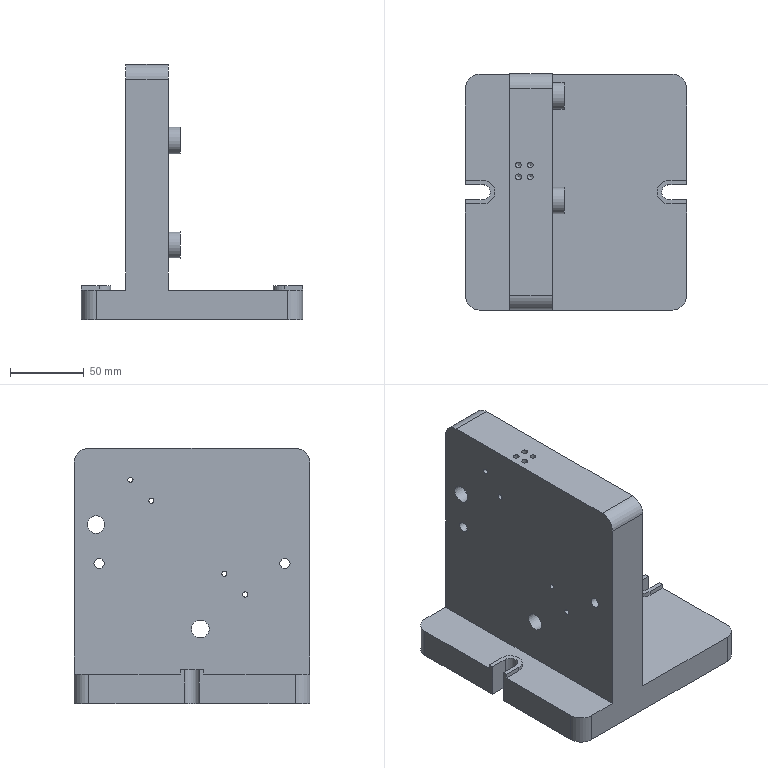Component | NX | FIXTURE_BODY | 1 solid | 52 faces | volume 1173446 mm3 | plane 24 | cylinder 24 | cone 4 | commonest cylinder face diameters 20 x6 3.5 x4 6.985 x2 18 x2 12 x2 10 x2 16 x2 3.838 x2